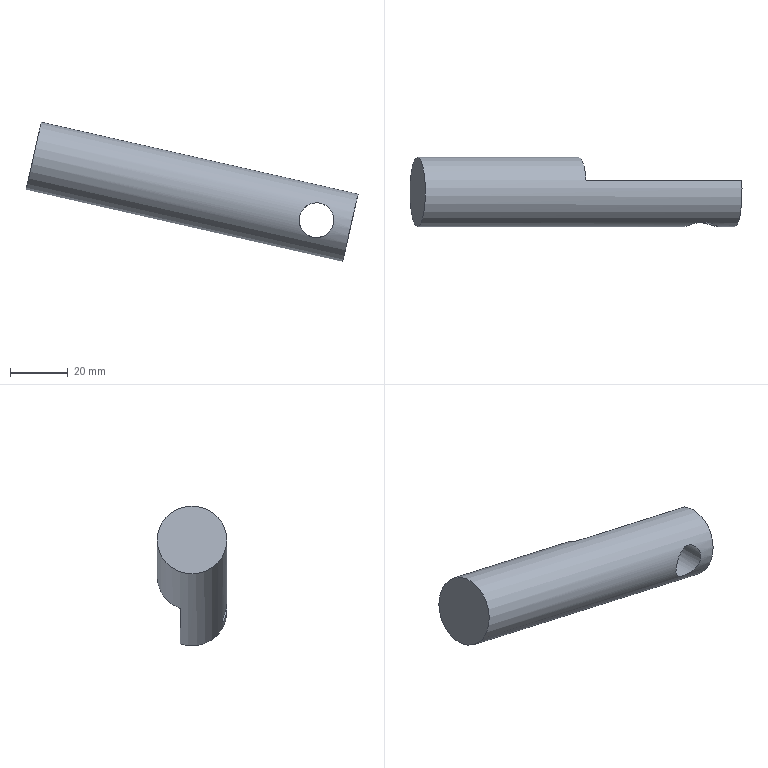Component | NX | SWING_ROD | 1 solid | 8 faces | box 114.53 x 24 x 48.22 mm | volume 41115 mm3 | plane 5 | cylinder 3 | commonest cylinder face diameters 12 x1 24 x1 16 x1
STEP:
#1=CARTESIAN_POINT('',(0.,0.,0.));
#2=DIRECTION('',(0.,0.,1.));
#3=DIRECTION('',(1.,0.,0.));
#4=AXIS2_PLACEMENT_3D('',#1,#2,#3);
#5=CARTESIAN_POINT('',(64.377,-12.,51.219));
#6=VERTEX_POINT('',#5);
#7=CARTESIAN_POINT('',(64.019,-12.,49.646));
#8=CARTESIAN_POINT('',(64.734,-12.,52.793));
#9=CARTESIAN_POINT('',(65.731,-11.635,54.15));
#10=CARTESIAN_POINT('',(68.334,-10.813,55.788));
#11=CARTESIAN_POINT('',(69.987,-10.394,56.094));
#12=CARTESIAN_POINT('',(73.1,-10.39,55.394));
#13=CARTESIAN_POINT('',(74.476,-10.81,54.398));
#14=CARTESIAN_POINT('',(76.121,-11.633,51.798));
#15=CARTESIAN_POINT('',(76.431,-11.998,50.13));
#16=CARTESIAN_POINT('',(75.734,-12.002,47.024));
#17=CARTESIAN_POINT('',(74.734,-11.639,45.639));
#18=CARTESIAN_POINT('',(72.122,-10.813,43.992));
#19=CARTESIAN_POINT('',(70.463,-10.395,43.688));
#20=CARTESIAN_POINT('',(67.363,-10.39,44.384));
#21=CARTESIAN_POINT('',(65.984,-10.808,45.374));
#22=CARTESIAN_POINT('',(64.328,-11.637,47.995));
#23=CARTESIAN_POINT('',(64.019,-12.,49.646));
#24=CARTESIAN_POINT('',(64.734,-12.,52.793));
#25=B_SPLINE_CURVE_WITH_KNOTS('',3,(#7,#8,#9,#10,#11,#12,#13,#14,#15,#16,#17,#18,#19,#20,#21,#22,#23,#24),.UNSPECIFIED.,.T.,.F.,(2,2,2,2,2,2,2,2,2,2,2),(-0.125,0.,0.125,0.25,0.375,0.5,0.625,0.75,0.875,1.,1.125),.UNSPECIFIED.);
#26=CARTESIAN_POINT('',(70.228,50.,49.89));
#27=DIRECTION('',(0.,-1.,0.));
#28=DIRECTION('',(-0.9752,0.,0.2215));
#29=AXIS2_PLACEMENT_3D('',#26,#27,#28);
#30=CYLINDRICAL_SURFACE('',#29,6.);
#31=CARTESIAN_POINT('',(6.283,62.));
#32=CARTESIAN_POINT('',(6.234,62.));
#33=CARTESIAN_POINT('',(6.137,61.976));
#34=CARTESIAN_POINT('',(5.993,61.879));
#35=CARTESIAN_POINT('',(5.85,61.732));
#36=CARTESIAN_POINT('',(5.708,61.548));
#37=CARTESIAN_POINT('',(5.567,61.338));
#38=CARTESIAN_POINT('',(5.428,61.111));
#39=CARTESIAN_POINT('',(5.287,60.891));
#40=CARTESIAN_POINT('',(5.145,60.693));
#41=CARTESIAN_POINT('',(5.003,60.531));
#42=CARTESIAN_POINT('',(4.859,60.421));
#43=CARTESIAN_POINT('',(4.715,60.378));
#44=CARTESIAN_POINT('',(4.57,60.419));
#45=CARTESIAN_POINT('',(4.426,60.528));
#46=CARTESIAN_POINT('',(4.283,60.69));
#47=CARTESIAN_POINT('',(4.14,60.888));
#48=CARTESIAN_POINT('',(3.999,61.108));
#49=CARTESIAN_POINT('',(3.859,61.335));
#50=CARTESIAN_POINT('',(3.718,61.546));
#51=CARTESIAN_POINT('',(3.576,61.73));
#52=CARTESIAN_POINT('',(3.432,61.877));
#53=CARTESIAN_POINT('',(3.289,61.975));
#54=CARTESIAN_POINT('',(3.144,62.012));
#55=CARTESIAN_POINT('',(3.,61.977));
#56=CARTESIAN_POINT('',(2.856,61.881));
#57=CARTESIAN_POINT('',(2.712,61.735));
#58=CARTESIAN_POINT('',(2.569,61.551));
#59=CARTESIAN_POINT('',(2.427,61.34));
#60=CARTESIAN_POINT('',(2.287,61.112));
#61=CARTESIAN_POINT('',(2.145,60.892));
#62=CARTESIAN_POINT('',(2.003,60.693));
#63=CARTESIAN_POINT('',(1.861,60.531));
#64=CARTESIAN_POINT('',(1.717,60.421));
#65=CARTESIAN_POINT('',(1.573,60.378));
#66=CARTESIAN_POINT('',(1.429,60.419));
#67=CARTESIAN_POINT('',(1.285,60.527));
#68=CARTESIAN_POINT('',(1.142,60.689));
#69=CARTESIAN_POINT('',(0.9992,60.887));
#70=CARTESIAN_POINT('',(0.8574,61.108));
#71=CARTESIAN_POINT('',(0.7166,61.337));
#72=CARTESIAN_POINT('',(0.5752,61.548));
#73=CARTESIAN_POINT('',(0.433,61.733));
#74=CARTESIAN_POINT('',(0.29,61.879));
#75=CARTESIAN_POINT('',(0.1459,61.976));
#76=CARTESIAN_POINT('',(0.04887,62.));
#77=CARTESIAN_POINT('',(-0.,62.));
#78=B_SPLINE_CURVE_WITH_KNOTS('',3,(#31,#32,#33,#34,#35,#36,#37,#38,#39,#40,#41,#42,#43,#44,#45,#46,#47,#48,#49,#50,#51,#52,#53,#54,#55,#56,#57,#58,#59,#60,#61,#62,#63,#64,#65,#66,#67,#68,#69,#70,#71,#72,#73,#74,#75,#76,#77),.UNSPECIFIED.,.F.,.F.,(4,1,1,1,1,1,1,1,1,1,1,1,1,1,1,1,1,1,1,1,1,1,1,1,1,1,1,1,1,1,1,1,1,1,1,1,1,1,1,1,1,1,1,1,4),(0.,0.02273,0.04545,0.06818,0.09091,0.1136,0.1364,0.1591,0.1818,0.2045,0.2273,0.25,0.2727,0.2955,0.3182,0.3409,0.3636,0.3864,0.4091,0.4318,0.4545,0.4773,0.5,0.5227,0.5455,0.5682,0.5909,0.6136,0.6364,0.6591,0.6818,0.7045,0.7273,0.75,0.7727,0.7955,0.8182,0.8409,0.8636,0.8864,0.9091,0.9318,0.9545,0.9773,1.),.QUASI_UNIFORM_KNOTS.);
#79=(GEOMETRIC_REPRESENTATION_CONTEXT(2)PARAMETRIC_REPRESENTATION_CONTEXT()REPRESENTATION_CONTEXT('',''));
#80=DEFINITIONAL_REPRESENTATION('',(#78),#79);
#81=PCURVE('',#30,#80);
#82=CARTESIAN_POINT('',(28.296,0.,59.417));
#83=DIRECTION('',(-0.9752,0.,0.2215));
#84=DIRECTION('',(0.,1.,0.));
#85=AXIS2_PLACEMENT_3D('',#82,#83,#84);
#86=CYLINDRICAL_SURFACE('',#85,12.);
#87=CARTESIAN_POINT('',(3.142,-37.));
#88=CARTESIAN_POINT('',(3.166,-37.));
#89=CARTESIAN_POINT('',(3.215,-37.044));
#90=CARTESIAN_POINT('',(3.285,-37.235));
#91=CARTESIAN_POINT('',(3.354,-37.54));
#92=CARTESIAN_POINT('',(3.418,-37.951));
#93=CARTESIAN_POINT('',(3.477,-38.459));
#94=CARTESIAN_POINT('',(3.53,-39.053));
#95=CARTESIAN_POINT('',(3.576,-39.731));
#96=CARTESIAN_POINT('',(3.614,-40.478));
#97=CARTESIAN_POINT('',(3.642,-41.279));
#98=CARTESIAN_POINT('',(3.661,-42.119));
#99=CARTESIAN_POINT('',(3.667,-42.986));
#100=CARTESIAN_POINT('',(3.661,-43.854));
#101=CARTESIAN_POINT('',(3.643,-44.698));
#102=CARTESIAN_POINT('',(3.614,-45.505));
#103=CARTESIAN_POINT('',(3.576,-46.257));
#104=CARTESIAN_POINT('',(3.53,-46.94));
#105=CARTESIAN_POINT('',(3.478,-47.535));
#106=CARTESIAN_POINT('',(3.418,-48.043));
#107=CARTESIAN_POINT('',(3.354,-48.455));
#108=CARTESIAN_POINT('',(3.286,-48.762));
#109=CARTESIAN_POINT('',(3.215,-48.953));
#110=CARTESIAN_POINT('',(3.143,-49.022));
#111=CARTESIAN_POINT('',(3.071,-48.958));
#112=CARTESIAN_POINT('',(3.,-48.769));
#113=CARTESIAN_POINT('',(2.931,-48.465));
#114=CARTESIAN_POINT('',(2.866,-48.055));
#115=CARTESIAN_POINT('',(2.807,-47.547));
#116=CARTESIAN_POINT('',(2.754,-46.951));
#117=CARTESIAN_POINT('',(2.707,-46.27));
#118=CARTESIAN_POINT('',(2.67,-45.521));
#119=CARTESIAN_POINT('',(2.641,-44.719));
#120=CARTESIAN_POINT('',(2.622,-43.879));
#121=CARTESIAN_POINT('',(2.616,-43.015));
#122=CARTESIAN_POINT('',(2.622,-42.15));
#123=CARTESIAN_POINT('',(2.64,-41.307));
#124=CARTESIAN_POINT('',(2.669,-40.5));
#125=CARTESIAN_POINT('',(2.707,-39.746));
#126=CARTESIAN_POINT('',(2.753,-39.06));
#127=CARTESIAN_POINT('',(2.806,-38.461));
#128=CARTESIAN_POINT('',(2.865,-37.951));
#129=CARTESIAN_POINT('',(2.93,-37.539));
#130=CARTESIAN_POINT('',(2.998,-37.234));
#131=CARTESIAN_POINT('',(3.069,-37.044));
#132=CARTESIAN_POINT('',(3.117,-37.));
#133=CARTESIAN_POINT('',(3.142,-37.));
#134=B_SPLINE_CURVE_WITH_KNOTS('',3,(#87,#88,#89,#90,#91,#92,#93,#94,#95,#96,#97,#98,#99,#100,#101,#102,#103,#104,#105,#106,#107,#108,#109,#110,#111,#112,#113,#114,#115,#116,#117,#118,#119,#120,#121,#122,#123,#124,#125,#126,#127,#128,#129,#130,#131,#132,#133),.UNSPECIFIED.,.T.,.F.,(4,1,1,1,1,1,1,1,1,1,1,1,1,1,1,1,1,1,1,1,1,1,1,1,1,1,1,1,1,1,1,1,1,1,1,1,1,1,1,1,1,1,1,1,4),(0.,0.02273,0.04545,0.06818,0.09091,0.1136,0.1364,0.1591,0.1818,0.2045,0.2273,0.25,0.2727,0.2955,0.3182,0.3409,0.3636,0.3864,0.4091,0.4318,0.4545,0.4773,0.5,0.5227,0.5455,0.5682,0.5909,0.6136,0.6364,0.6591,0.6818,0.7045,0.7273,0.75,0.7727,0.7955,0.8182,0.8409,0.8636,0.8864,0.9091,0.9318,0.9545,0.9773,1.),.QUASI_UNIFORM_KNOTS.);
#135=(GEOMETRIC_REPRESENTATION_CONTEXT(2)PARAMETRIC_REPRESENTATION_CONTEXT()REPRESENTATION_CONTEXT('',''));
#136=DEFINITIONAL_REPRESENTATION('',(#134),#135);
#137=PCURVE('',#86,#136);
#138=SURFACE_CURVE('',#25,(#81,#137),.PCURVE_S1.);
#139=EDGE_CURVE('',#6,#6,#138,.T.);
#140=ORIENTED_EDGE('',*,*,#139,.T.);
#141=CARTESIAN_POINT('',(64.377,-2.,51.219));
#142=VERTEX_POINT('',#141);
#143=CARTESIAN_POINT('',(64.377,-2.,51.219));
#144=CARTESIAN_POINT('',(64.377,-12.,51.219));
#145=B_SPLINE_CURVE_WITH_KNOTS('',1,(#143,#144),.UNSPECIFIED.,.F.,.F.,(2,2),(52.,62.),.PIECEWISE_BEZIER_KNOTS.);
#146=CARTESIAN_POINT('',(-0.,0.));
#147=DIRECTION('',(0.,1.));
#148=VECTOR('',#147,1.);
#149=LINE('',#146,#148);
#150=(GEOMETRIC_REPRESENTATION_CONTEXT(2)PARAMETRIC_REPRESENTATION_CONTEXT()REPRESENTATION_CONTEXT('',''));
#151=DEFINITIONAL_REPRESENTATION('',(#149),#150);
#152=PCURVE('',#30,#151);
#153=CARTESIAN_POINT('',(6.283,0.));
#154=DIRECTION('',(0.,1.));
#155=VECTOR('',#154,1.);
#156=LINE('',#153,#155);
#157=(GEOMETRIC_REPRESENTATION_CONTEXT(2)PARAMETRIC_REPRESENTATION_CONTEXT()REPRESENTATION_CONTEXT('',''));
#158=DEFINITIONAL_REPRESENTATION('',(#156),#157);
#159=PCURVE('',#30,#158);
#160=SEAM_CURVE('',#145,(#152,#159),.PCURVE_S1.);
#161=EDGE_CURVE('',#142,#6,#160,.T.);
#162=ORIENTED_EDGE('',*,*,#161,.F.);
#163=CARTESIAN_POINT('',(70.228,-2.,49.89));
#164=DIRECTION('',(0.,-1.,0.));
#165=DIRECTION('',(-0.9752,0.,0.2215));
#166=AXIS2_PLACEMENT_3D('',#163,#164,#165);
#167=CIRCLE('',#166,6.);
#168=CARTESIAN_POINT('',(0.,52.));
#169=DIRECTION('',(1.,0.));
#170=VECTOR('',#169,1.);
#171=LINE('',#168,#170);
#172=(GEOMETRIC_REPRESENTATION_CONTEXT(2)PARAMETRIC_REPRESENTATION_CONTEXT()REPRESENTATION_CONTEXT('',''));
#173=DEFINITIONAL_REPRESENTATION('',(#171),#172);
#174=PCURVE('',#30,#173);
#175=CARTESIAN_POINT('',(70.228,-2.,49.89));
#176=DIRECTION('',(0.,1.,0.));
#177=DIRECTION('',(0.9752,0.,-0.2215));
#178=AXIS2_PLACEMENT_3D('',#175,#176,#177);
#179=PLANE('',#178);
#180=CARTESIAN_POINT('',(-6.,0.));
#181=CARTESIAN_POINT('',(-6.,10.392));
#182=CARTESIAN_POINT('',(3.,5.196));
#183=CARTESIAN_POINT('',(12.,0.));
#184=CARTESIAN_POINT('',(3.,-5.196));
#185=CARTESIAN_POINT('',(-6.,-10.392));
#186=CARTESIAN_POINT('',(-6.,0.));
#187=(BOUNDED_CURVE()B_SPLINE_CURVE(2,(#180,#181,#182,#183,#184,#185,#186),.UNSPECIFIED.,.T.,.F.)B_SPLINE_CURVE_WITH_KNOTS((1,2,2,2,2,1),(-2.094,0.,2.094,4.189,6.283,8.378),.UNSPECIFIED.)CURVE()GEOMETRIC_REPRESENTATION_ITEM()RATIONAL_B_SPLINE_CURVE((1.,0.5,1.,0.5,1.,0.5,1.))REPRESENTATION_ITEM(''));
#188=(GEOMETRIC_REPRESENTATION_CONTEXT(2)PARAMETRIC_REPRESENTATION_CONTEXT()REPRESENTATION_CONTEXT('',''));
#189=DEFINITIONAL_REPRESENTATION('',(#187),#188);
#190=PCURVE('',#179,#189);
#191=SURFACE_CURVE('',#167,(#174,#190),.PCURVE_S1.);
#192=EDGE_CURVE('',#142,#142,#191,.T.);
#193=ORIENTED_EDGE('',*,*,#192,.T.);
#194=ORIENTED_EDGE('',*,*,#161,.T.);
#195=EDGE_LOOP('',(#140,#162,#193,#194));
#196=FACE_BOUND('',#195,.F.);
#197=ADVANCED_FACE('',(#196),#30,.F.);
#198=CARTESIAN_POINT('',(79.423,4.,36.199));
#199=VERTEX_POINT('',#198);
#200=CARTESIAN_POINT('',(25.79,4.,48.384));
#201=VERTEX_POINT('',#200);
#202=CARTESIAN_POINT('',(25.79,4.,48.384));
#203=DIRECTION('',(-0.9752,0.,0.2215));
#204=VECTOR('',#203,1.);
#205=LINE('',#202,#204);
#206=CARTESIAN_POINT('',(1.231,0.));
#207=DIRECTION('',(0.,1.));
#208=VECTOR('',#207,1.);
#209=LINE('',#206,#208);
#210=(GEOMETRIC_REPRESENTATION_CONTEXT(2)PARAMETRIC_REPRESENTATION_CONTEXT()REPRESENTATION_CONTEXT('',''));
#211=DEFINITIONAL_REPRESENTATION('',(#209),#210);
#212=PCURVE('',#86,#211);
#213=CARTESIAN_POINT('',(30.803,4.,70.449));
#214=DIRECTION('',(0.,-1.,0.));
#215=DIRECTION('',(-0.9752,0.,0.2215));
#216=AXIS2_PLACEMENT_3D('',#213,#214,#215);
#217=PLANE('',#216);
#218=CARTESIAN_POINT('',(0.,22.627));
#219=DIRECTION('',(1.,0.));
#220=VECTOR('',#219,1.);
#221=LINE('',#218,#220);
#222=(GEOMETRIC_REPRESENTATION_CONTEXT(2)PARAMETRIC_REPRESENTATION_CONTEXT()REPRESENTATION_CONTEXT('',''));
#223=DEFINITIONAL_REPRESENTATION('',(#221),#222);
#224=PCURVE('',#217,#223);
#225=SURFACE_CURVE('',#205,(#212,#224),.PCURVE_S1.);
#226=EDGE_CURVE('',#199,#201,#225,.T.);
#227=ORIENTED_EDGE('',*,*,#226,.F.);
#228=CARTESIAN_POINT('',(84.436,4.,58.264));
#229=VERTEX_POINT('',#228);
#230=CARTESIAN_POINT('',(81.93,0.,47.232));
#231=DIRECTION('',(-0.9752,0.,0.2215));
#232=DIRECTION('',(0.,1.,0.));
#233=AXIS2_PLACEMENT_3D('',#230,#231,#232);
#234=CIRCLE('',#233,12.);
#235=CARTESIAN_POINT('',(0.,-55.));
#236=DIRECTION('',(1.,-0.));
#237=VECTOR('',#236,1.);
#238=LINE('',#235,#237);
#239=(GEOMETRIC_REPRESENTATION_CONTEXT(2)PARAMETRIC_REPRESENTATION_CONTEXT()REPRESENTATION_CONTEXT('',''));
#240=DEFINITIONAL_REPRESENTATION('',(#238),#239);
#241=PCURVE('',#86,#240);
#242=CARTESIAN_POINT('',(79.271,0.,35.53));
#243=DIRECTION('',(0.9752,0.,-0.2215));
#244=DIRECTION('',(0.,-1.,0.));
#245=AXIS2_PLACEMENT_3D('',#242,#243,#244);
#246=PLANE('',#245);
#247=CARTESIAN_POINT('',(-12.,-12.));
#248=CARTESIAN_POINT('',(-12.,8.785));
#249=CARTESIAN_POINT('',(6.,-1.608));
#250=CARTESIAN_POINT('',(24.,-12.));
#251=CARTESIAN_POINT('',(6.,-22.392));
#252=CARTESIAN_POINT('',(-12.,-32.785));
#253=CARTESIAN_POINT('',(-12.,-12.));
#254=(BOUNDED_CURVE()B_SPLINE_CURVE(2,(#247,#248,#249,#250,#251,#252,#253),.UNSPECIFIED.,.T.,.F.)B_SPLINE_CURVE_WITH_KNOTS((1,2,2,2,2,1),(-2.094,0.,2.094,4.189,6.283,8.378),.UNSPECIFIED.)CURVE()GEOMETRIC_REPRESENTATION_ITEM()RATIONAL_B_SPLINE_CURVE((1.,0.5,1.,0.5,1.,0.5,1.))REPRESENTATION_ITEM(''));
#255=(GEOMETRIC_REPRESENTATION_CONTEXT(2)PARAMETRIC_REPRESENTATION_CONTEXT()REPRESENTATION_CONTEXT('',''));
#256=DEFINITIONAL_REPRESENTATION('',(#254),#255);
#257=PCURVE('',#246,#256);
#258=SURFACE_CURVE('',#234,(#241,#257),.PCURVE_S1.);
#259=EDGE_CURVE('',#199,#229,#258,.T.);
#260=ORIENTED_EDGE('',*,*,#259,.T.);
#261=CARTESIAN_POINT('',(30.803,4.,70.449));
#262=VERTEX_POINT('',#261);
#263=CARTESIAN_POINT('',(30.803,4.,70.449));
#264=DIRECTION('',(0.9752,0.,-0.2215));
#265=VECTOR('',#264,1.);
#266=LINE('',#263,#265);
#267=CARTESIAN_POINT('',(5.052,-0.));
#268=DIRECTION('',(0.,-1.));
#269=VECTOR('',#268,1.);
#270=LINE('',#267,#269);
#271=(GEOMETRIC_REPRESENTATION_CONTEXT(2)PARAMETRIC_REPRESENTATION_CONTEXT()REPRESENTATION_CONTEXT('',''));
#272=DEFINITIONAL_REPRESENTATION('',(#270),#271);
#273=PCURVE('',#86,#272);
#274=CARTESIAN_POINT('',(0.,0.));
#275=DIRECTION('',(-1.,0.));
#276=VECTOR('',#275,1.);
#277=LINE('',#274,#276);
#278=(GEOMETRIC_REPRESENTATION_CONTEXT(2)PARAMETRIC_REPRESENTATION_CONTEXT()REPRESENTATION_CONTEXT('',''));
#279=DEFINITIONAL_REPRESENTATION('',(#277),#278);
#280=PCURVE('',#217,#279);
#281=SURFACE_CURVE('',#266,(#273,#280),.PCURVE_S1.);
#282=EDGE_CURVE('',#262,#229,#281,.T.);
#283=ORIENTED_EDGE('',*,*,#282,.F.);
#284=CARTESIAN_POINT('',(28.296,12.,59.417));
#285=VERTEX_POINT('',#284);
#286=CARTESIAN_POINT('',(28.296,0.,59.417));
#287=DIRECTION('',(0.9752,0.,-0.2215));
#288=DIRECTION('',(0.,1.,0.));
#289=AXIS2_PLACEMENT_3D('',#286,#287,#288);
#290=CIRCLE('',#289,12.);
#291=CARTESIAN_POINT('',(12.566,-0.));
#292=DIRECTION('',(-1.,0.));
#293=VECTOR('',#292,1.);
#294=LINE('',#291,#293);
#295=(GEOMETRIC_REPRESENTATION_CONTEXT(2)PARAMETRIC_REPRESENTATION_CONTEXT()REPRESENTATION_CONTEXT('',''));
#296=DEFINITIONAL_REPRESENTATION('',(#294),#295);
#297=PCURVE('',#86,#296);
#298=CARTESIAN_POINT('',(28.296,0.,59.417));
#299=DIRECTION('',(0.9752,0.,-0.2215));
#300=DIRECTION('',(0.,-1.,0.));
#301=AXIS2_PLACEMENT_3D('',#298,#299,#300);
#302=PLANE('',#301);
#303=CARTESIAN_POINT('',(0.,0.));
#304=DIRECTION('',(-1.,0.));
#305=AXIS2_PLACEMENT_2D('',#303,#304);
#306=CIRCLE('',#305,12.);
#307=(GEOMETRIC_REPRESENTATION_CONTEXT(2)PARAMETRIC_REPRESENTATION_CONTEXT()REPRESENTATION_CONTEXT('',''));
#308=DEFINITIONAL_REPRESENTATION('',(#306),#307);
#309=PCURVE('',#302,#308);
#310=SURFACE_CURVE('',#290,(#297,#309),.PCURVE_S1.);
#311=EDGE_CURVE('',#285,#262,#310,.T.);
#312=ORIENTED_EDGE('',*,*,#311,.F.);
#313=CARTESIAN_POINT('',(-27.287,12.,72.045));
#314=VERTEX_POINT('',#313);
#315=CARTESIAN_POINT('',(28.296,12.,59.417));
#316=CARTESIAN_POINT('',(-27.287,12.,72.045));
#317=B_SPLINE_CURVE_WITH_KNOTS('',1,(#315,#316),.UNSPECIFIED.,.F.,.F.,(2,2),(0.,57.),.PIECEWISE_BEZIER_KNOTS.);
#318=CARTESIAN_POINT('',(6.283,0.));
#319=DIRECTION('',(0.,1.));
#320=VECTOR('',#319,1.);
#321=LINE('',#318,#320);
#322=(GEOMETRIC_REPRESENTATION_CONTEXT(2)PARAMETRIC_REPRESENTATION_CONTEXT()REPRESENTATION_CONTEXT('',''));
#323=DEFINITIONAL_REPRESENTATION('',(#321),#322);
#324=PCURVE('',#86,#323);
#325=CARTESIAN_POINT('',(0.,0.));
#326=DIRECTION('',(0.,1.));
#327=VECTOR('',#326,1.);
#328=LINE('',#325,#327);
#329=(GEOMETRIC_REPRESENTATION_CONTEXT(2)PARAMETRIC_REPRESENTATION_CONTEXT()REPRESENTATION_CONTEXT('',''));
#330=DEFINITIONAL_REPRESENTATION('',(#328),#329);
#331=PCURVE('',#86,#330);
#332=SEAM_CURVE('',#317,(#324,#331),.PCURVE_S1.);
#333=EDGE_CURVE('',#285,#314,#332,.T.);
#334=ORIENTED_EDGE('',*,*,#333,.T.);
#335=CARTESIAN_POINT('',(-27.287,0.,72.045));
#336=DIRECTION('',(-0.9752,0.,0.2215));
#337=DIRECTION('',(0.,1.,0.));
#338=AXIS2_PLACEMENT_3D('',#335,#336,#337);
#339=CIRCLE('',#338,12.);
#340=CARTESIAN_POINT('',(0.,57.));
#341=DIRECTION('',(1.,0.));
#342=VECTOR('',#341,1.);
#343=LINE('',#340,#342);
#344=(GEOMETRIC_REPRESENTATION_CONTEXT(2)PARAMETRIC_REPRESENTATION_CONTEXT()REPRESENTATION_CONTEXT('',''));
#345=DEFINITIONAL_REPRESENTATION('',(#343),#344);
#346=PCURVE('',#86,#345);
#347=CARTESIAN_POINT('',(-27.287,0.,72.045));
#348=DIRECTION('',(-0.9752,0.,0.2215));
#349=DIRECTION('',(0.,1.,0.));
#350=AXIS2_PLACEMENT_3D('',#347,#348,#349);
#351=PLANE('',#350);
#352=CARTESIAN_POINT('',(0.,0.));
#353=DIRECTION('',(1.,0.));
#354=AXIS2_PLACEMENT_2D('',#352,#353);
#355=CIRCLE('',#354,12.);
#356=(GEOMETRIC_REPRESENTATION_CONTEXT(2)PARAMETRIC_REPRESENTATION_CONTEXT()REPRESENTATION_CONTEXT('',''));
#357=DEFINITIONAL_REPRESENTATION('',(#355),#356);
#358=PCURVE('',#351,#357);
#359=SURFACE_CURVE('',#339,(#346,#358),.PCURVE_S1.);
#360=EDGE_CURVE('',#314,#314,#359,.T.);
#361=ORIENTED_EDGE('',*,*,#360,.F.);
#362=ORIENTED_EDGE('',*,*,#333,.F.);
#363=CARTESIAN_POINT('',(28.296,0.,59.417));
#364=DIRECTION('',(0.9752,0.,-0.2215));
#365=DIRECTION('',(0.,1.,0.));
#366=AXIS2_PLACEMENT_3D('',#363,#364,#365);
#367=CIRCLE('',#366,12.);
#368=CARTESIAN_POINT('',(6.283,-0.));
#369=DIRECTION('',(-1.,0.));
#370=VECTOR('',#369,1.);
#371=LINE('',#368,#370);
#372=(GEOMETRIC_REPRESENTATION_CONTEXT(2)PARAMETRIC_REPRESENTATION_CONTEXT()REPRESENTATION_CONTEXT('',''));
#373=DEFINITIONAL_REPRESENTATION('',(#371),#372);
#374=PCURVE('',#86,#373);
#375=CARTESIAN_POINT('',(0.,0.));
#376=DIRECTION('',(-1.,0.));
#377=AXIS2_PLACEMENT_2D('',#375,#376);
#378=CIRCLE('',#377,12.);
#379=(GEOMETRIC_REPRESENTATION_CONTEXT(2)PARAMETRIC_REPRESENTATION_CONTEXT()REPRESENTATION_CONTEXT('',''));
#380=DEFINITIONAL_REPRESENTATION('',(#378),#379);
#381=PCURVE('',#302,#380);
#382=SURFACE_CURVE('',#367,(#374,#381),.PCURVE_S1.);
#383=EDGE_CURVE('',#201,#285,#382,.T.);
#384=ORIENTED_EDGE('',*,*,#383,.F.);
#385=EDGE_LOOP('',(#227,#260,#283,#312,#334,#361,#362,#384));
#386=FACE_BOUND('',#385,.T.);
#387=ORIENTED_EDGE('',*,*,#139,.T.);
#388=EDGE_LOOP('',(#387));
#389=FACE_BOUND('',#388,.T.);
#390=ADVANCED_FACE('',(#386,#389),#86,.T.);
#391=CARTESIAN_POINT('',(84.436,4.,58.264));
#392=DIRECTION('',(-0.2215,0.,-0.9752));
#393=VECTOR('',#392,1.);
#394=LINE('',#391,#393);
#395=CARTESIAN_POINT('',(-4.,-23.314));
#396=DIRECTION('',(0.,1.));
#397=VECTOR('',#396,1.);
#398=LINE('',#395,#397);
#399=(GEOMETRIC_REPRESENTATION_CONTEXT(2)PARAMETRIC_REPRESENTATION_CONTEXT()REPRESENTATION_CONTEXT('',''));
#400=DEFINITIONAL_REPRESENTATION('',(#398),#399);
#401=PCURVE('',#246,#400);
#402=CARTESIAN_POINT('',(-55.,-0.));
#403=DIRECTION('',(0.,1.));
#404=VECTOR('',#403,1.);
#405=LINE('',#402,#404);
#406=(GEOMETRIC_REPRESENTATION_CONTEXT(2)PARAMETRIC_REPRESENTATION_CONTEXT()REPRESENTATION_CONTEXT('',''));
#407=DEFINITIONAL_REPRESENTATION('',(#405),#406);
#408=PCURVE('',#217,#407);
#409=SURFACE_CURVE('',#394,(#401,#408),.PCURVE_S1.);
#410=EDGE_CURVE('',#229,#199,#409,.T.);
#411=ORIENTED_EDGE('',*,*,#410,.F.);
#412=ORIENTED_EDGE('',*,*,#259,.F.);
#413=EDGE_LOOP('',(#411,#412));
#414=FACE_BOUND('',#413,.T.);
#415=ADVANCED_FACE('',(#414),#246,.T.);
#416=ORIENTED_EDGE('',*,*,#360,.T.);
#417=EDGE_LOOP('',(#416));
#418=FACE_BOUND('',#417,.T.);
#419=ADVANCED_FACE('',(#418),#351,.T.);
#420=CARTESIAN_POINT('',(62.427,4.,51.663));
#421=VERTEX_POINT('',#420);
#422=CARTESIAN_POINT('',(70.228,4.,49.89));
#423=DIRECTION('',(0.,1.,0.));
#424=DIRECTION('',(-0.9752,0.,0.2215));
#425=AXIS2_PLACEMENT_3D('',#422,#423,#424);
#426=CIRCLE('',#425,8.);
#427=CARTESIAN_POINT('',(-35.,11.314));
#428=CARTESIAN_POINT('',(-35.,-2.543));
#429=CARTESIAN_POINT('',(-47.,4.386));
#430=CARTESIAN_POINT('',(-59.,11.314));
#431=CARTESIAN_POINT('',(-47.,18.242));
#432=CARTESIAN_POINT('',(-35.,25.17));
#433=CARTESIAN_POINT('',(-35.,11.314));
#434=(BOUNDED_CURVE()B_SPLINE_CURVE(2,(#427,#428,#429,#430,#431,#432,#433),.UNSPECIFIED.,.T.,.F.)B_SPLINE_CURVE_WITH_KNOTS((1,2,2,2,2,1),(-2.094,0.,2.094,4.189,6.283,8.378),.UNSPECIFIED.)CURVE()GEOMETRIC_REPRESENTATION_ITEM()RATIONAL_B_SPLINE_CURVE((1.,0.5,1.,0.5,1.,0.5,1.))REPRESENTATION_ITEM(''));
#435=(GEOMETRIC_REPRESENTATION_CONTEXT(2)PARAMETRIC_REPRESENTATION_CONTEXT()REPRESENTATION_CONTEXT('',''));
#436=DEFINITIONAL_REPRESENTATION('',(#434),#435);
#437=PCURVE('',#217,#436);
#438=CARTESIAN_POINT('',(70.228,-2.,49.89));
#439=DIRECTION('',(0.,1.,0.));
#440=DIRECTION('',(0.9752,0.,-0.2215));
#441=AXIS2_PLACEMENT_3D('',#438,#439,#440);
#442=CYLINDRICAL_SURFACE('',#441,8.);
#443=CARTESIAN_POINT('',(3.142,6.));
#444=DIRECTION('',(1.,0.));
#445=VECTOR('',#444,1.);
#446=LINE('',#443,#445);
#447=(GEOMETRIC_REPRESENTATION_CONTEXT(2)PARAMETRIC_REPRESENTATION_CONTEXT()REPRESENTATION_CONTEXT('',''));
#448=DEFINITIONAL_REPRESENTATION('',(#446),#447);
#449=PCURVE('',#442,#448);
#450=SURFACE_CURVE('',#426,(#437,#449),.PCURVE_S1.);
#451=EDGE_CURVE('',#421,#421,#450,.T.);
#452=ORIENTED_EDGE('',*,*,#451,.F.);
#453=EDGE_LOOP('',(#452));
#454=FACE_BOUND('',#453,.T.);
#455=ORIENTED_EDGE('',*,*,#410,.T.);
#456=ORIENTED_EDGE('',*,*,#226,.T.);
#457=CARTESIAN_POINT('',(30.803,4.,70.449));
#458=DIRECTION('',(0.2215,0.,0.9752));
#459=VECTOR('',#458,1.);
#460=LINE('',#457,#459);
#461=CARTESIAN_POINT('',(0.,0.));
#462=DIRECTION('',(0.,-1.));
#463=VECTOR('',#462,1.);
#464=LINE('',#461,#463);
#465=(GEOMETRIC_REPRESENTATION_CONTEXT(2)PARAMETRIC_REPRESENTATION_CONTEXT()REPRESENTATION_CONTEXT('',''));
#466=DEFINITIONAL_REPRESENTATION('',(#464),#465);
#467=PCURVE('',#217,#466);
#468=CARTESIAN_POINT('',(-4.,-11.314));
#469=DIRECTION('',(0.,-1.));
#470=VECTOR('',#469,1.);
#471=LINE('',#468,#470);
#472=(GEOMETRIC_REPRESENTATION_CONTEXT(2)PARAMETRIC_REPRESENTATION_CONTEXT()REPRESENTATION_CONTEXT('',''));
#473=DEFINITIONAL_REPRESENTATION('',(#471),#472);
#474=PCURVE('',#302,#473);
#475=SURFACE_CURVE('',#460,(#467,#474),.PCURVE_S1.);
#476=EDGE_CURVE('',#201,#262,#475,.T.);
#477=ORIENTED_EDGE('',*,*,#476,.T.);
#478=ORIENTED_EDGE('',*,*,#282,.T.);
#479=EDGE_LOOP('',(#455,#456,#477,#478));
#480=FACE_BOUND('',#479,.T.);
#481=ADVANCED_FACE('',(#454,#480),#217,.F.);
#482=ORIENTED_EDGE('',*,*,#383,.T.);
#483=ORIENTED_EDGE('',*,*,#311,.T.);
#484=ORIENTED_EDGE('',*,*,#476,.F.);
#485=EDGE_LOOP('',(#482,#483,#484));
#486=FACE_BOUND('',#485,.T.);
#487=ADVANCED_FACE('',(#486),#302,.T.);
#488=CARTESIAN_POINT('',(62.427,-2.,51.663));
#489=VERTEX_POINT('',#488);
#490=CARTESIAN_POINT('',(70.228,-2.,49.89));
#491=DIRECTION('',(0.,-1.,0.));
#492=DIRECTION('',(-0.9752,0.,0.2215));
#493=AXIS2_PLACEMENT_3D('',#490,#491,#492);
#494=CIRCLE('',#493,8.);
#495=CARTESIAN_POINT('',(9.425,0.));
#496=DIRECTION('',(-1.,0.));
#497=VECTOR('',#496,1.);
#498=LINE('',#495,#497);
#499=(GEOMETRIC_REPRESENTATION_CONTEXT(2)PARAMETRIC_REPRESENTATION_CONTEXT()REPRESENTATION_CONTEXT('',''));
#500=DEFINITIONAL_REPRESENTATION('',(#498),#499);
#501=PCURVE('',#442,#500);
#502=CARTESIAN_POINT('',(-8.,0.));
#503=CARTESIAN_POINT('',(-8.,13.856));
#504=CARTESIAN_POINT('',(4.,6.928));
#505=CARTESIAN_POINT('',(16.,-0.));
#506=CARTESIAN_POINT('',(4.,-6.928));
#507=CARTESIAN_POINT('',(-8.,-13.856));
#508=CARTESIAN_POINT('',(-8.,0.));
#509=(BOUNDED_CURVE()B_SPLINE_CURVE(2,(#502,#503,#504,#505,#506,#507,#508),.UNSPECIFIED.,.T.,.F.)B_SPLINE_CURVE_WITH_KNOTS((1,2,2,2,2,1),(-2.094,0.,2.094,4.189,6.283,8.378),.UNSPECIFIED.)CURVE()GEOMETRIC_REPRESENTATION_ITEM()RATIONAL_B_SPLINE_CURVE((1.,0.5,1.,0.5,1.,0.5,1.))REPRESENTATION_ITEM(''));
#510=(GEOMETRIC_REPRESENTATION_CONTEXT(2)PARAMETRIC_REPRESENTATION_CONTEXT()REPRESENTATION_CONTEXT('',''));
#511=DEFINITIONAL_REPRESENTATION('',(#509),#510);
#512=PCURVE('',#179,#511);
#513=SURFACE_CURVE('',#494,(#501,#512),.PCURVE_S1.);
#514=EDGE_CURVE('',#489,#489,#513,.T.);
#515=ORIENTED_EDGE('',*,*,#514,.F.);
#516=CARTESIAN_POINT('',(62.427,-2.,51.663));
#517=CARTESIAN_POINT('',(62.427,4.,51.663));
#518=B_SPLINE_CURVE_WITH_KNOTS('',1,(#516,#517),.UNSPECIFIED.,.F.,.F.,(2,2),(0.,6.),.PIECEWISE_BEZIER_KNOTS.);
#519=CARTESIAN_POINT('',(9.425,0.));
#520=DIRECTION('',(0.,1.));
#521=VECTOR('',#520,1.);
#522=LINE('',#519,#521);
#523=(GEOMETRIC_REPRESENTATION_CONTEXT(2)PARAMETRIC_REPRESENTATION_CONTEXT()REPRESENTATION_CONTEXT('',''));
#524=DEFINITIONAL_REPRESENTATION('',(#522),#523);
#525=PCURVE('',#442,#524);
#526=CARTESIAN_POINT('',(3.142,0.));
#527=DIRECTION('',(0.,1.));
#528=VECTOR('',#527,1.);
#529=LINE('',#526,#528);
#530=(GEOMETRIC_REPRESENTATION_CONTEXT(2)PARAMETRIC_REPRESENTATION_CONTEXT()REPRESENTATION_CONTEXT('',''));
#531=DEFINITIONAL_REPRESENTATION('',(#529),#530);
#532=PCURVE('',#442,#531);
#533=SEAM_CURVE('',#518,(#525,#532),.PCURVE_S1.);
#534=EDGE_CURVE('',#489,#421,#533,.T.);
#535=ORIENTED_EDGE('',*,*,#534,.T.);
#536=ORIENTED_EDGE('',*,*,#451,.F.);
#537=ORIENTED_EDGE('',*,*,#534,.F.);
#538=EDGE_LOOP('',(#515,#535,#536,#537));
#539=FACE_BOUND('',#538,.F.);
#540=ADVANCED_FACE('',(#539),#442,.F.);
#541=ORIENTED_EDGE('',*,*,#514,.F.);
#542=EDGE_LOOP('',(#541));
#543=FACE_BOUND('',#542,.T.);
#544=ORIENTED_EDGE('',*,*,#192,.T.);
#545=EDGE_LOOP('',(#544));
#546=FACE_BOUND('',#545,.T.);
#547=ADVANCED_FACE('',(#543,#546),#179,.T.);
#548=CLOSED_SHELL('',(#197,#390,#415,#419,#481,#487,#540,#547));
#549=MANIFOLD_SOLID_BREP('',#548);
#550=(LENGTH_UNIT()NAMED_UNIT(*)SI_UNIT(.MILLI.,.METRE.));
#551=UNCERTAINTY_MEASURE_WITH_UNIT(LENGTH_MEASURE(0.0005),#550,'','');
#552=(NAMED_UNIT(*)PLANE_ANGLE_UNIT()SI_UNIT($,.RADIAN.));
#553=(NAMED_UNIT(*)SI_UNIT($,.STERADIAN.)SOLID_ANGLE_UNIT());
#554=(GEOMETRIC_REPRESENTATION_CONTEXT(3)GLOBAL_UNCERTAINTY_ASSIGNED_CONTEXT((#551))GLOBAL_UNIT_ASSIGNED_CONTEXT((#550,#552,#553))REPRESENTATION_CONTEXT('',''));
#555=ADVANCED_BREP_SHAPE_REPRESENTATION('',(#4,#549),#554);